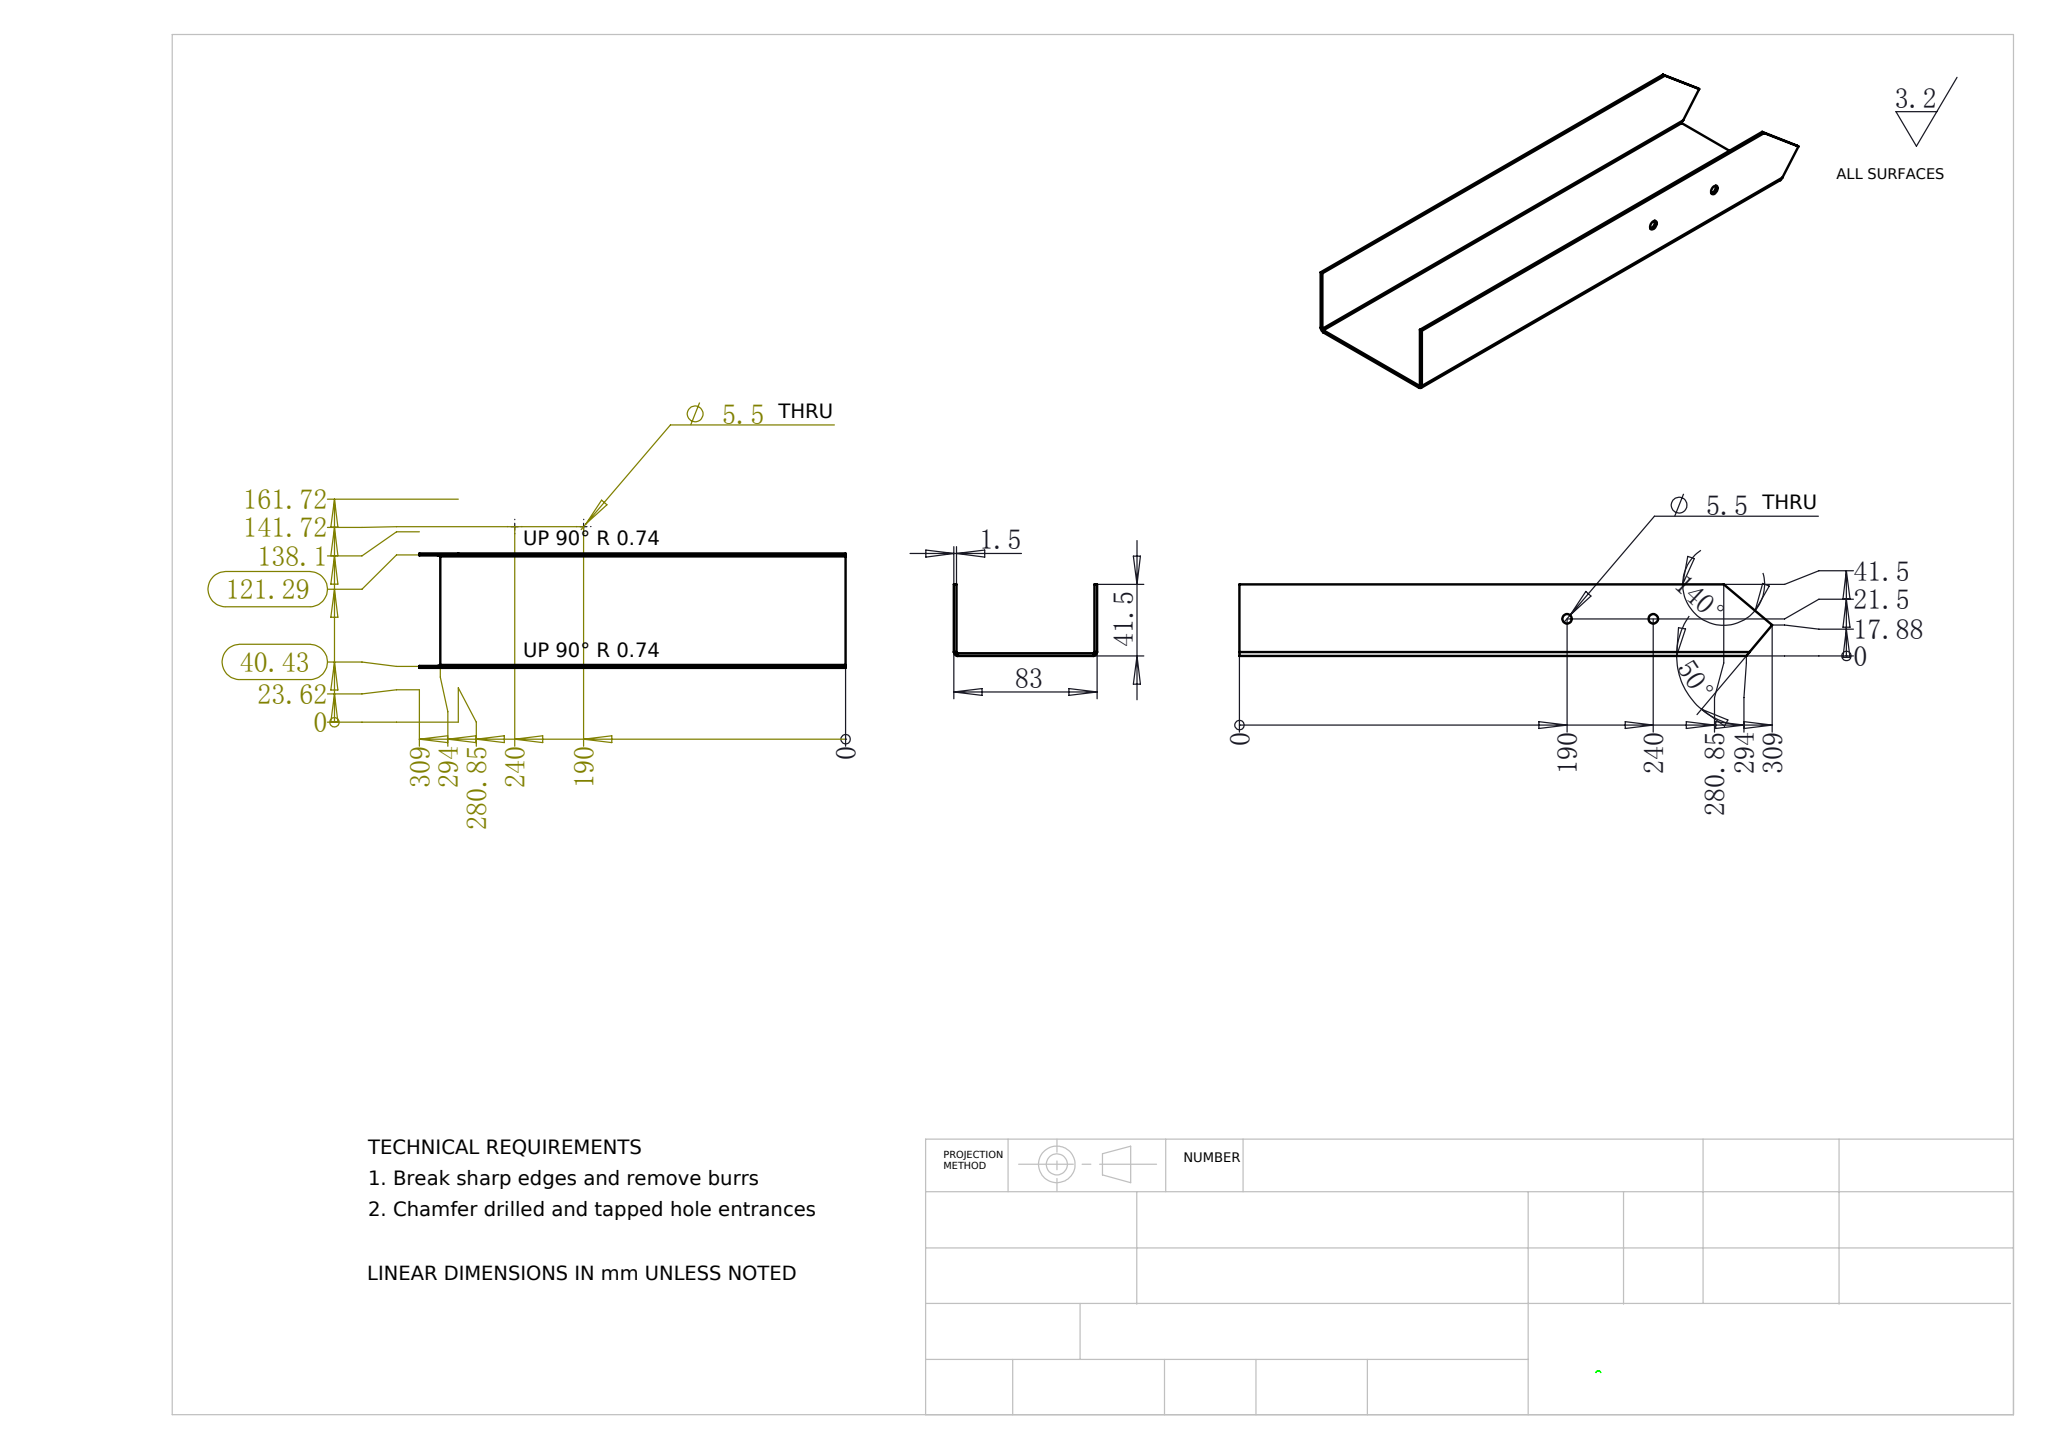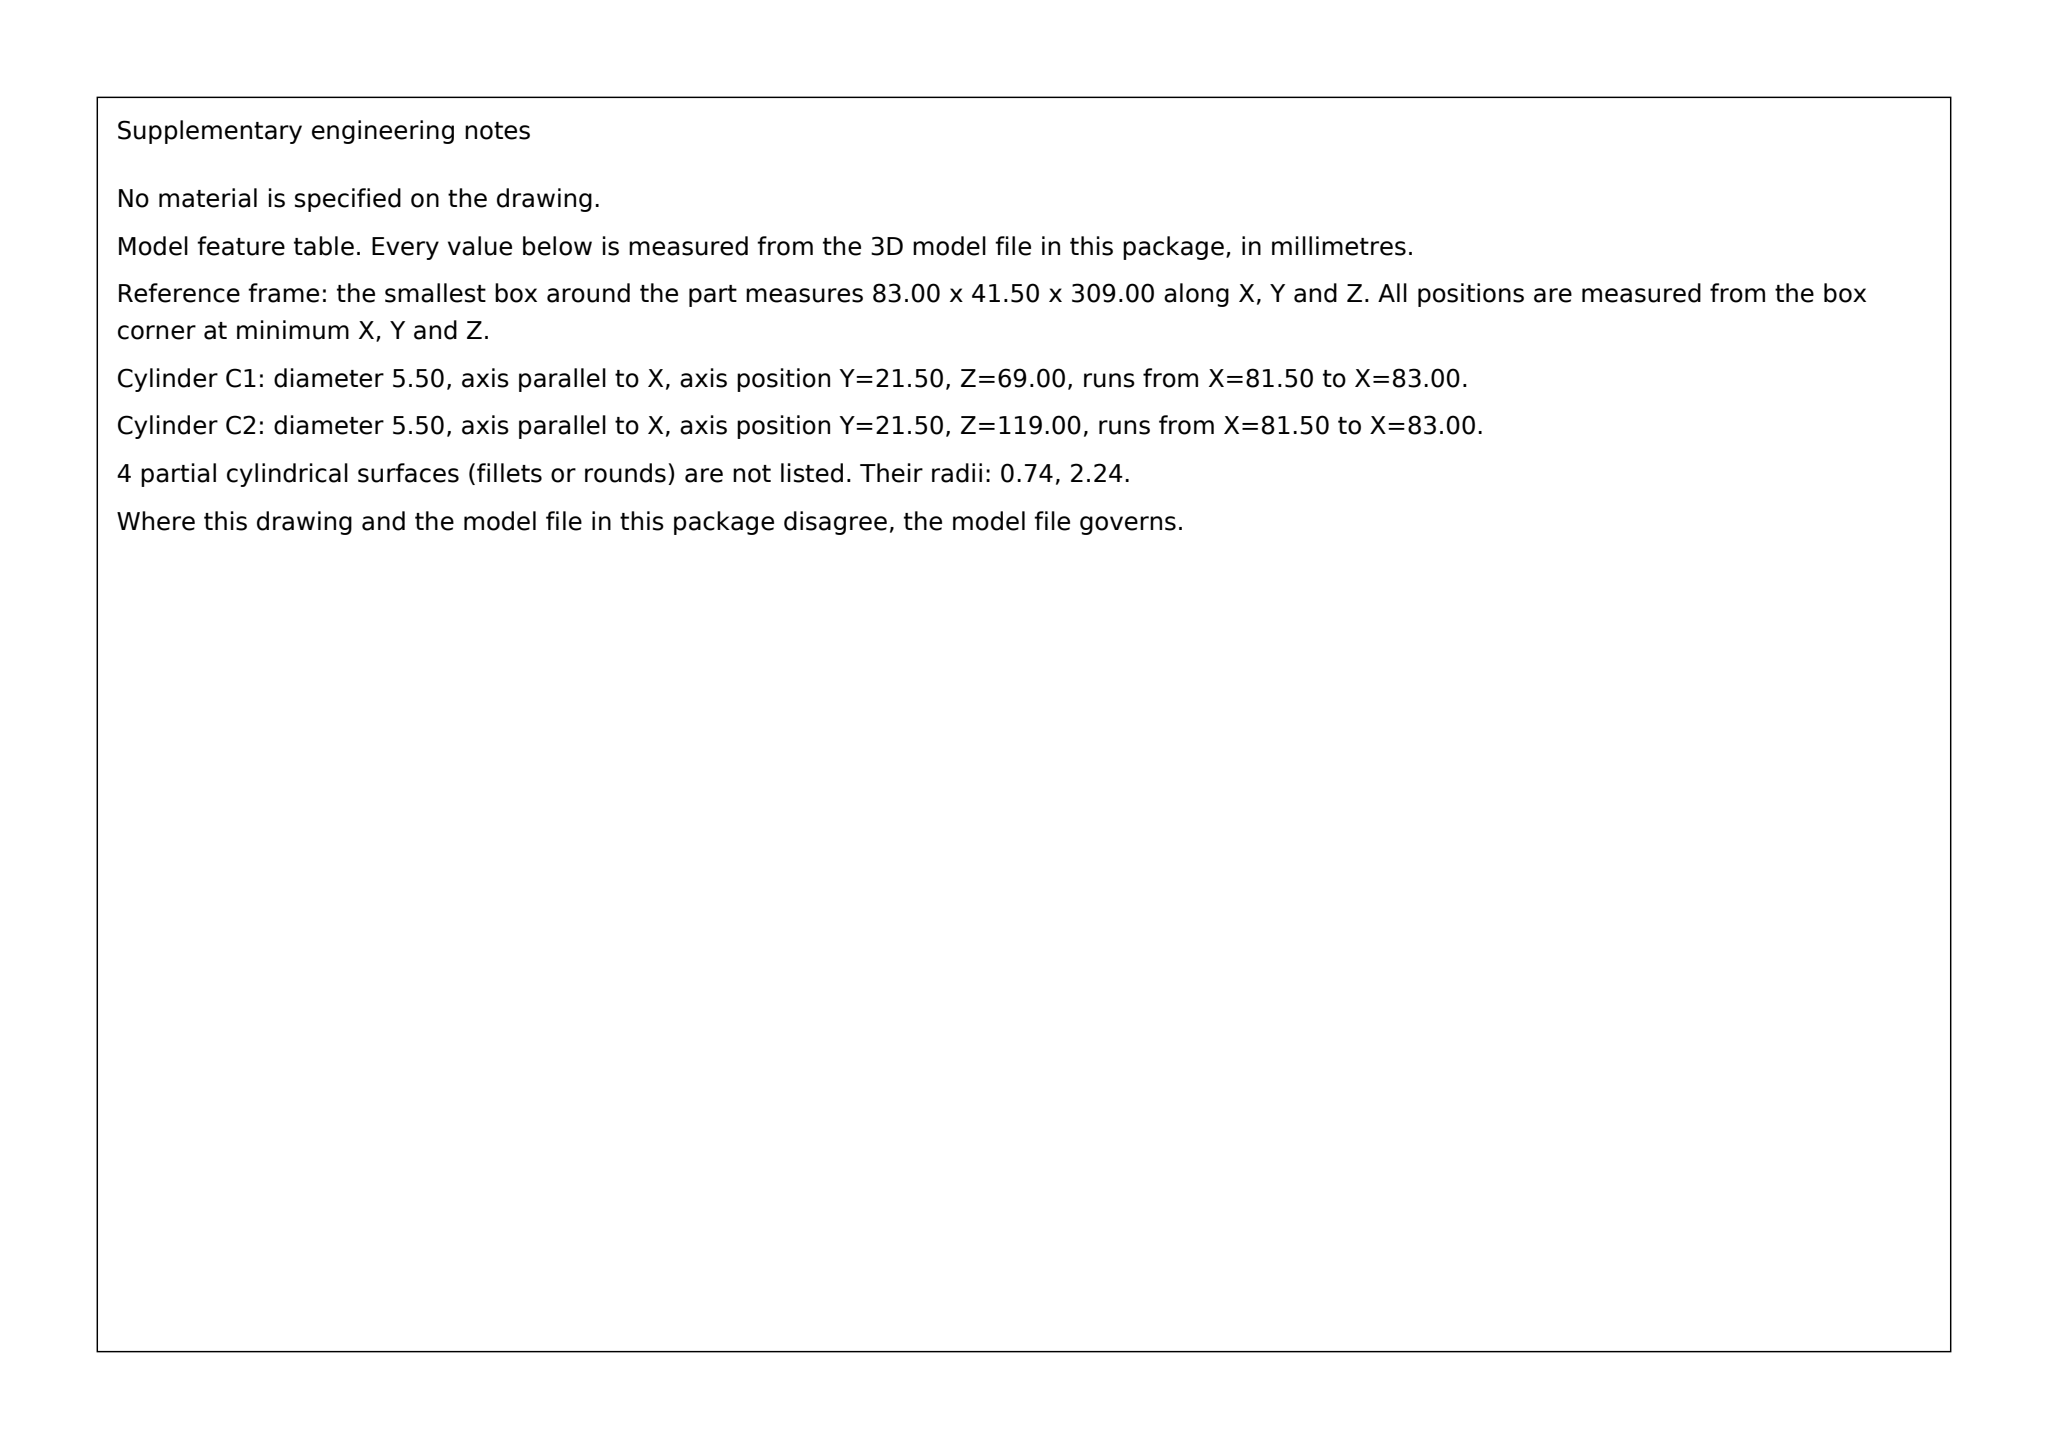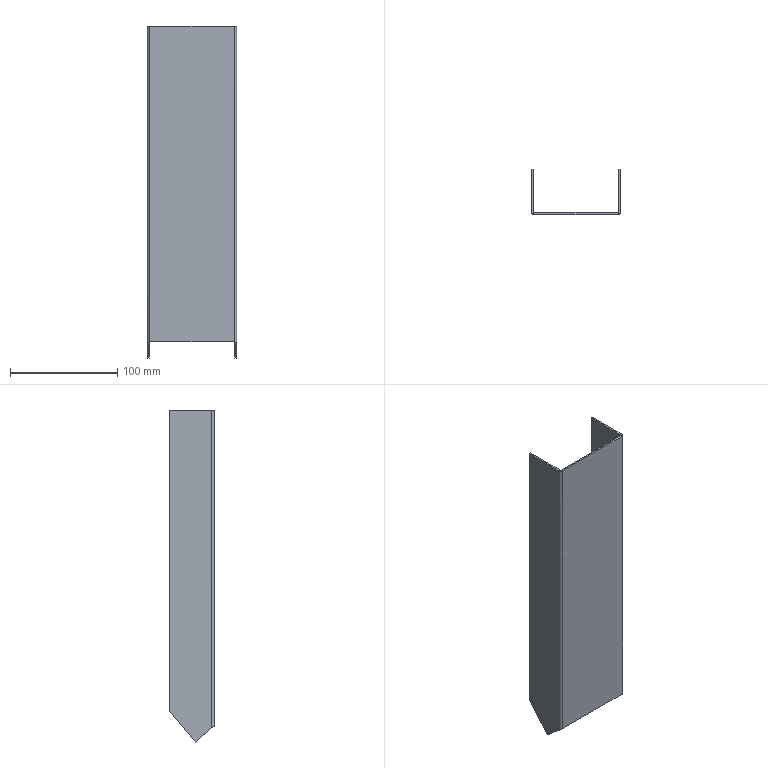Part | SolidWorks | mm | 1 solid | 28 faces | box 83 x 41.5 x 309 mm | volume 71715 mm3 | plane 18 | cylinder 8 | spline 2 | commonest cylinder face diameters 5.5 x4 1.473 x2 4.473 x2
STEP:
#1=CARTESIAN_POINT('',(80.,20.,-232.75));
#2=VERTEX_POINT('',#1);
#3=CARTESIAN_POINT('',(80.,20.,-227.25));
#4=VERTEX_POINT('',#3);
#5=CARTESIAN_POINT('',(80.,20.,-230.));
#6=DIRECTION('',(-1.,0.,0.));
#7=DIRECTION('',(0.,0.,1.));
#8=AXIS2_PLACEMENT_3D('',#5,#6,#7);
#9=CIRCLE('',#8,2.75);
#10=EDGE_CURVE('',#2,#4,#9,.T.);
#11=ORIENTED_EDGE('',*,*,#10,.T.);
#12=CARTESIAN_POINT('',(81.5,20.,-227.25));
#13=VERTEX_POINT('',#12);
#14=CARTESIAN_POINT('',(81.5,20.,-227.25));
#15=DIRECTION('',(1.,0.,0.));
#16=VECTOR('',#15,1000.);
#17=LINE('',#14,#16);
#18=EDGE_CURVE('',#4,#13,#17,.T.);
#19=ORIENTED_EDGE('',*,*,#18,.T.);
#20=CARTESIAN_POINT('',(81.5,20.,-232.75));
#21=VERTEX_POINT('',#20);
#22=CARTESIAN_POINT('',(81.5,20.,-230.));
#23=DIRECTION('',(1.,0.,0.));
#24=DIRECTION('',(0.,0.,-1.));
#25=AXIS2_PLACEMENT_3D('',#22,#23,#24);
#26=CIRCLE('',#25,2.75);
#27=EDGE_CURVE('',#13,#21,#26,.T.);
#28=ORIENTED_EDGE('',*,*,#27,.T.);
#29=CARTESIAN_POINT('',(81.5,20.,-232.75));
#30=DIRECTION('',(1.,0.,0.));
#31=VECTOR('',#30,1000.);
#32=LINE('',#29,#31);
#33=EDGE_CURVE('',#2,#21,#32,.T.);
#34=ORIENTED_EDGE('',*,*,#33,.F.);
#35=EDGE_LOOP('',(#11,#19,#28,#34));
#36=FACE_OUTER_BOUND('',#35,.T.);
#37=CARTESIAN_POINT('',(81.5,20.,-230.));
#38=DIRECTION('',(1.,0.,0.));
#39=DIRECTION('',(0.,0.,-1.));
#40=AXIS2_PLACEMENT_3D('',#37,#38,#39);
#41=CYLINDRICAL_SURFACE('',#40,2.75);
#42=ADVANCED_FACE('',(#36),#41,.F.);
#43=CARTESIAN_POINT('',(80.,20.,-182.75));
#44=VERTEX_POINT('',#43);
#45=CARTESIAN_POINT('',(80.,20.,-177.25));
#46=VERTEX_POINT('',#45);
#47=CARTESIAN_POINT('',(80.,20.,-180.));
#48=DIRECTION('',(-1.,0.,0.));
#49=DIRECTION('',(0.,0.,1.));
#50=AXIS2_PLACEMENT_3D('',#47,#48,#49);
#51=CIRCLE('',#50,2.75);
#52=EDGE_CURVE('',#44,#46,#51,.T.);
#53=ORIENTED_EDGE('',*,*,#52,.T.);
#54=CARTESIAN_POINT('',(81.5,20.,-177.25));
#55=VERTEX_POINT('',#54);
#56=CARTESIAN_POINT('',(81.5,20.,-177.25));
#57=DIRECTION('',(1.,0.,0.));
#58=VECTOR('',#57,1000.);
#59=LINE('',#56,#58);
#60=EDGE_CURVE('',#46,#55,#59,.T.);
#61=ORIENTED_EDGE('',*,*,#60,.T.);
#62=CARTESIAN_POINT('',(81.5,20.,-182.75));
#63=VERTEX_POINT('',#62);
#64=CARTESIAN_POINT('',(81.5,20.,-180.));
#65=DIRECTION('',(1.,0.,0.));
#66=DIRECTION('',(0.,0.,-1.));
#67=AXIS2_PLACEMENT_3D('',#64,#65,#66);
#68=CIRCLE('',#67,2.75);
#69=EDGE_CURVE('',#55,#63,#68,.T.);
#70=ORIENTED_EDGE('',*,*,#69,.T.);
#71=CARTESIAN_POINT('',(81.5,20.,-182.75));
#72=DIRECTION('',(1.,0.,0.));
#73=VECTOR('',#72,1000.);
#74=LINE('',#71,#73);
#75=EDGE_CURVE('',#44,#63,#74,.T.);
#76=ORIENTED_EDGE('',*,*,#75,.F.);
#77=EDGE_LOOP('',(#53,#61,#70,#76));
#78=FACE_OUTER_BOUND('',#77,.T.);
#79=CARTESIAN_POINT('',(81.5,20.,-180.));
#80=DIRECTION('',(1.,0.,0.));
#81=DIRECTION('',(0.,0.,-1.));
#82=AXIS2_PLACEMENT_3D('',#79,#80,#81);
#83=CYLINDRICAL_SURFACE('',#82,2.75);
#84=ADVANCED_FACE('',(#78),#83,.F.);
#85=CARTESIAN_POINT('',(81.5,20.,-230.));
#86=DIRECTION('',(1.,0.,0.));
#87=DIRECTION('',(0.,0.,-1.));
#88=AXIS2_PLACEMENT_3D('',#85,#86,#87);
#89=CIRCLE('',#88,2.75);
#90=EDGE_CURVE('',#21,#13,#89,.T.);
#91=ORIENTED_EDGE('',*,*,#90,.F.);
#92=ORIENTED_EDGE('',*,*,#27,.F.);
#93=EDGE_LOOP('',(#91,#92));
#94=FACE_BOUND('',#93,.T.);
#95=CARTESIAN_POINT('',(81.5,20.,-180.));
#96=DIRECTION('',(1.,0.,0.));
#97=DIRECTION('',(0.,0.,-1.));
#98=AXIS2_PLACEMENT_3D('',#95,#96,#97);
#99=CIRCLE('',#98,2.75);
#100=EDGE_CURVE('',#63,#55,#99,.T.);
#101=ORIENTED_EDGE('',*,*,#100,.F.);
#102=ORIENTED_EDGE('',*,*,#69,.F.);
#103=EDGE_LOOP('',(#101,#102));
#104=FACE_BOUND('',#103,.T.);
#105=CARTESIAN_POINT('',(81.5,0.7366,-285.877));
#106=VERTEX_POINT('',#105);
#107=CARTESIAN_POINT('',(81.5,16.376,-299.));
#108=VERTEX_POINT('',#107);
#109=CARTESIAN_POINT('',(81.5,-145.387,-163.265));
#110=DIRECTION('',(0.,0.766,-0.6428));
#111=VECTOR('',#110,1000.);
#112=LINE('',#109,#111);
#113=EDGE_CURVE('',#106,#108,#112,.T.);
#114=ORIENTED_EDGE('',*,*,#113,.T.);
#115=CARTESIAN_POINT('',(81.5,40.,-270.846));
#116=VERTEX_POINT('',#115);
#117=CARTESIAN_POINT('',(81.5,161.763,-125.735));
#118=DIRECTION('',(0.,0.6428,0.766));
#119=VECTOR('',#118,1000.);
#120=LINE('',#117,#119);
#121=EDGE_CURVE('',#108,#116,#120,.T.);
#122=ORIENTED_EDGE('',*,*,#121,.T.);
#123=CARTESIAN_POINT('',(81.5,40.,10.));
#124=VERTEX_POINT('',#123);
#125=CARTESIAN_POINT('',(81.5,40.,10.));
#126=DIRECTION('',(0.,0.,-1.));
#127=VECTOR('',#126,1000.);
#128=LINE('',#125,#127);
#129=EDGE_CURVE('',#124,#116,#128,.T.);
#130=ORIENTED_EDGE('',*,*,#129,.F.);
#131=CARTESIAN_POINT('',(81.5,0.7366,10.));
#132=VERTEX_POINT('',#131);
#133=CARTESIAN_POINT('',(81.5,0.,10.));
#134=DIRECTION('',(0.,1.,0.));
#135=VECTOR('',#134,1000.);
#136=LINE('',#133,#135);
#137=EDGE_CURVE('',#132,#124,#136,.T.);
#138=ORIENTED_EDGE('',*,*,#137,.F.);
#139=CARTESIAN_POINT('',(81.5,0.7366,10.));
#140=DIRECTION('',(0.,0.,-1.));
#141=VECTOR('',#140,1000.);
#142=LINE('',#139,#141);
#143=EDGE_CURVE('',#132,#106,#142,.T.);
#144=ORIENTED_EDGE('',*,*,#143,.T.);
#145=EDGE_LOOP('',(#114,#122,#130,#138,#144));
#146=FACE_OUTER_BOUND('',#145,.T.);
#147=CARTESIAN_POINT('',(81.5,0.,10.));
#148=DIRECTION('',(-1.,0.,0.));
#149=DIRECTION('',(0.,0.,1.));
#150=AXIS2_PLACEMENT_3D('',#147,#148,#149);
#151=PLANE('',#150);
#152=ADVANCED_FACE('',(#94,#104,#146),#151,.F.);
#153=ORIENTED_EDGE('',*,*,#129,.T.);
#154=CARTESIAN_POINT('',(80.,40.,-270.846));
#155=VERTEX_POINT('',#154);
#156=CARTESIAN_POINT('',(80.,40.,-270.846));
#157=DIRECTION('',(1.,0.,0.));
#158=VECTOR('',#157,1000.);
#159=LINE('',#156,#158);
#160=EDGE_CURVE('',#155,#116,#159,.T.);
#161=ORIENTED_EDGE('',*,*,#160,.F.);
#162=CARTESIAN_POINT('',(80.,40.,10.));
#163=VERTEX_POINT('',#162);
#164=CARTESIAN_POINT('',(80.,40.,10.));
#165=DIRECTION('',(0.,0.,-1.));
#166=VECTOR('',#165,1000.);
#167=LINE('',#164,#166);
#168=EDGE_CURVE('',#163,#155,#167,.T.);
#169=ORIENTED_EDGE('',*,*,#168,.F.);
#170=CARTESIAN_POINT('',(80.,40.,10.));
#171=DIRECTION('',(1.,0.,0.));
#172=VECTOR('',#171,1000.);
#173=LINE('',#170,#172);
#174=EDGE_CURVE('',#163,#124,#173,.T.);
#175=ORIENTED_EDGE('',*,*,#174,.T.);
#176=EDGE_LOOP('',(#153,#161,#169,#175));
#177=FACE_OUTER_BOUND('',#176,.T.);
#178=CARTESIAN_POINT('',(80.,40.,10.));
#179=DIRECTION('',(0.,1.,0.));
#180=DIRECTION('',(0.,0.,1.));
#181=AXIS2_PLACEMENT_3D('',#178,#179,#180);
#182=PLANE('',#181);
#183=ADVANCED_FACE('',(#177),#182,.T.);
#184=ORIENTED_EDGE('',*,*,#10,.F.);
#185=CARTESIAN_POINT('',(80.,20.,-230.));
#186=DIRECTION('',(-1.,0.,0.));
#187=DIRECTION('',(0.,0.,1.));
#188=AXIS2_PLACEMENT_3D('',#185,#186,#187);
#189=CIRCLE('',#188,2.75);
#190=EDGE_CURVE('',#4,#2,#189,.T.);
#191=ORIENTED_EDGE('',*,*,#190,.F.);
#192=EDGE_LOOP('',(#184,#191));
#193=FACE_BOUND('',#192,.T.);
#194=ORIENTED_EDGE('',*,*,#52,.F.);
#195=CARTESIAN_POINT('',(80.,20.,-180.));
#196=DIRECTION('',(-1.,0.,0.));
#197=DIRECTION('',(0.,0.,1.));
#198=AXIS2_PLACEMENT_3D('',#195,#196,#197);
#199=CIRCLE('',#198,2.75);
#200=EDGE_CURVE('',#46,#44,#199,.T.);
#201=ORIENTED_EDGE('',*,*,#200,.F.);
#202=EDGE_LOOP('',(#194,#201));
#203=FACE_BOUND('',#202,.T.);
#204=CARTESIAN_POINT('',(80.,16.376,-299.));
#205=VERTEX_POINT('',#204);
#206=CARTESIAN_POINT('',(80.,161.763,-125.735));
#207=DIRECTION('',(0.,0.6428,0.766));
#208=VECTOR('',#207,1000.);
#209=LINE('',#206,#208);
#210=EDGE_CURVE('',#205,#155,#209,.T.);
#211=ORIENTED_EDGE('',*,*,#210,.F.);
#212=CARTESIAN_POINT('',(80.,0.7366,-285.877));
#213=VERTEX_POINT('',#212);
#214=CARTESIAN_POINT('',(80.,-145.387,-163.265));
#215=DIRECTION('',(0.,0.766,-0.6428));
#216=VECTOR('',#215,1000.);
#217=LINE('',#214,#216);
#218=EDGE_CURVE('',#213,#205,#217,.T.);
#219=ORIENTED_EDGE('',*,*,#218,.F.);
#220=CARTESIAN_POINT('',(80.,0.7366,10.));
#221=VERTEX_POINT('',#220);
#222=CARTESIAN_POINT('',(80.,0.7366,10.));
#223=DIRECTION('',(0.,0.,-1.));
#224=VECTOR('',#223,1000.);
#225=LINE('',#222,#224);
#226=EDGE_CURVE('',#221,#213,#225,.T.);
#227=ORIENTED_EDGE('',*,*,#226,.F.);
#228=CARTESIAN_POINT('',(80.,0.,10.));
#229=DIRECTION('',(0.,1.,0.));
#230=VECTOR('',#229,1000.);
#231=LINE('',#228,#230);
#232=EDGE_CURVE('',#221,#163,#231,.T.);
#233=ORIENTED_EDGE('',*,*,#232,.T.);
#234=ORIENTED_EDGE('',*,*,#168,.T.);
#235=EDGE_LOOP('',(#211,#219,#227,#233,#234));
#236=FACE_OUTER_BOUND('',#235,.T.);
#237=CARTESIAN_POINT('',(80.,0.,10.));
#238=DIRECTION('',(-1.,0.,0.));
#239=DIRECTION('',(0.,0.,1.));
#240=AXIS2_PLACEMENT_3D('',#237,#238,#239);
#241=PLANE('',#240);
#242=ADVANCED_FACE('',(#193,#203,#236),#241,.T.);
#243=ORIENTED_EDGE('',*,*,#226,.T.);
#244=CARTESIAN_POINT('',(79.263,0.,-284.));
#245=VERTEX_POINT('',#244);
#246=CARTESIAN_POINT('',(79.263,0.,-284.));
#247=CARTESIAN_POINT('',(79.695,-0.,-284.));
#248=CARTESIAN_POINT('',(80.,0.3051,-284.777));
#249=CARTESIAN_POINT('',(80.,0.7366,-285.877));
#250=(BOUNDED_CURVE()B_SPLINE_CURVE(3,(#246,#247,#248,#249),.UNSPECIFIED.,.F.,.F.)B_SPLINE_CURVE_WITH_KNOTS((4,4),(3.142,4.712),.UNSPECIFIED.)CURVE()GEOMETRIC_REPRESENTATION_ITEM()RATIONAL_B_SPLINE_CURVE((1.,0.8047,0.8047,1.))REPRESENTATION_ITEM(''));
#251=EDGE_CURVE('',#245,#213,#250,.T.);
#252=ORIENTED_EDGE('',*,*,#251,.F.);
#253=CARTESIAN_POINT('',(79.263,0.,10.));
#254=VERTEX_POINT('',#253);
#255=CARTESIAN_POINT('',(79.263,0.,10.));
#256=DIRECTION('',(0.,0.,-1.));
#257=VECTOR('',#256,1000.);
#258=LINE('',#255,#257);
#259=EDGE_CURVE('',#254,#245,#258,.T.);
#260=ORIENTED_EDGE('',*,*,#259,.F.);
#261=CARTESIAN_POINT('',(79.263,0.7366,10.));
#262=DIRECTION('',(0.,0.,1.));
#263=DIRECTION('',(-1.,0.,0.));
#264=AXIS2_PLACEMENT_3D('',#261,#262,#263);
#265=CIRCLE('',#264,0.7366);
#266=EDGE_CURVE('',#254,#221,#265,.T.);
#267=ORIENTED_EDGE('',*,*,#266,.T.);
#268=EDGE_LOOP('',(#243,#252,#260,#267));
#269=FACE_OUTER_BOUND('',#268,.T.);
#270=CARTESIAN_POINT('',(79.263,0.7366,10.));
#271=DIRECTION('',(0.,0.,-1.));
#272=DIRECTION('',(-1.,0.,0.));
#273=AXIS2_PLACEMENT_3D('',#270,#271,#272);
#274=CYLINDRICAL_SURFACE('',#273,0.7366);
#275=ADVANCED_FACE('',(#269),#274,.F.);
#276=ORIENTED_EDGE('',*,*,#259,.T.);
#277=CARTESIAN_POINT('',(0.7366,0.,-284.));
#278=VERTEX_POINT('',#277);
#279=CARTESIAN_POINT('',(0.,0.,-284.));
#280=DIRECTION('',(-1.,0.,0.));
#281=VECTOR('',#280,1000.);
#282=LINE('',#279,#281);
#283=EDGE_CURVE('',#245,#278,#282,.T.);
#284=ORIENTED_EDGE('',*,*,#283,.T.);
#285=CARTESIAN_POINT('',(0.7366,0.,10.));
#286=VERTEX_POINT('',#285);
#287=CARTESIAN_POINT('',(0.7366,0.,10.));
#288=DIRECTION('',(0.,0.,-1.));
#289=VECTOR('',#288,1000.);
#290=LINE('',#287,#289);
#291=EDGE_CURVE('',#286,#278,#290,.T.);
#292=ORIENTED_EDGE('',*,*,#291,.F.);
#293=CARTESIAN_POINT('',(0.,0.,10.));
#294=DIRECTION('',(1.,0.,0.));
#295=VECTOR('',#294,1000.);
#296=LINE('',#293,#295);
#297=EDGE_CURVE('',#286,#254,#296,.T.);
#298=ORIENTED_EDGE('',*,*,#297,.T.);
#299=EDGE_LOOP('',(#276,#284,#292,#298));
#300=FACE_OUTER_BOUND('',#299,.T.);
#301=CARTESIAN_POINT('',(0.,0.,10.));
#302=DIRECTION('',(0.,1.,0.));
#303=DIRECTION('',(0.,0.,1.));
#304=AXIS2_PLACEMENT_3D('',#301,#302,#303);
#305=PLANE('',#304);
#306=ADVANCED_FACE('',(#300),#305,.T.);
#307=ORIENTED_EDGE('',*,*,#291,.T.);
#308=CARTESIAN_POINT('',(0.,0.7366,-285.877));
#309=VERTEX_POINT('',#308);
#310=CARTESIAN_POINT('',(0.,0.7366,-285.877));
#311=CARTESIAN_POINT('',(-0.,0.3051,-284.777));
#312=CARTESIAN_POINT('',(0.3051,-0.,-284.));
#313=CARTESIAN_POINT('',(0.7366,0.,-284.));
#314=(BOUNDED_CURVE()B_SPLINE_CURVE(3,(#310,#311,#312,#313),.UNSPECIFIED.,.F.,.F.)B_SPLINE_CURVE_WITH_KNOTS((4,4),(1.571,3.142),.UNSPECIFIED.)CURVE()GEOMETRIC_REPRESENTATION_ITEM()RATIONAL_B_SPLINE_CURVE((1.,0.8047,0.8047,1.))REPRESENTATION_ITEM(''));
#315=EDGE_CURVE('',#309,#278,#314,.T.);
#316=ORIENTED_EDGE('',*,*,#315,.F.);
#317=CARTESIAN_POINT('',(0.,0.7366,10.));
#318=VERTEX_POINT('',#317);
#319=CARTESIAN_POINT('',(0.,0.7366,10.));
#320=DIRECTION('',(0.,0.,-1.));
#321=VECTOR('',#320,1000.);
#322=LINE('',#319,#321);
#323=EDGE_CURVE('',#318,#309,#322,.T.);
#324=ORIENTED_EDGE('',*,*,#323,.F.);
#325=CARTESIAN_POINT('',(0.7366,0.7366,10.));
#326=DIRECTION('',(0.,0.,1.));
#327=DIRECTION('',(-1.,0.,0.));
#328=AXIS2_PLACEMENT_3D('',#325,#326,#327);
#329=CIRCLE('',#328,0.7366);
#330=EDGE_CURVE('',#318,#286,#329,.T.);
#331=ORIENTED_EDGE('',*,*,#330,.T.);
#332=EDGE_LOOP('',(#307,#316,#324,#331));
#333=FACE_OUTER_BOUND('',#332,.T.);
#334=CARTESIAN_POINT('',(0.7366,0.7366,10.));
#335=DIRECTION('',(0.,0.,-1.));
#336=DIRECTION('',(-1.,0.,0.));
#337=AXIS2_PLACEMENT_3D('',#334,#335,#336);
#338=CYLINDRICAL_SURFACE('',#337,0.7366);
#339=ADVANCED_FACE('',(#333),#338,.F.);
#340=CARTESIAN_POINT('',(0.,16.376,-299.));
#341=VERTEX_POINT('',#340);
#342=CARTESIAN_POINT('',(0.,-145.387,-163.265));
#343=DIRECTION('',(0.,-0.766,0.6428));
#344=VECTOR('',#343,1000.);
#345=LINE('',#342,#344);
#346=EDGE_CURVE('',#341,#309,#345,.T.);
#347=ORIENTED_EDGE('',*,*,#346,.F.);
#348=CARTESIAN_POINT('',(0.,40.,-270.846));
#349=VERTEX_POINT('',#348);
#350=CARTESIAN_POINT('',(0.,161.763,-125.735));
#351=DIRECTION('',(0.,-0.6428,-0.766));
#352=VECTOR('',#351,1000.);
#353=LINE('',#350,#352);
#354=EDGE_CURVE('',#349,#341,#353,.T.);
#355=ORIENTED_EDGE('',*,*,#354,.F.);
#356=CARTESIAN_POINT('',(0.,40.,10.));
#357=VERTEX_POINT('',#356);
#358=CARTESIAN_POINT('',(0.,40.,10.));
#359=DIRECTION('',(0.,0.,-1.));
#360=VECTOR('',#359,1000.);
#361=LINE('',#358,#360);
#362=EDGE_CURVE('',#357,#349,#361,.T.);
#363=ORIENTED_EDGE('',*,*,#362,.F.);
#364=CARTESIAN_POINT('',(0.,0.,10.));
#365=DIRECTION('',(0.,-1.,0.));
#366=VECTOR('',#365,1000.);
#367=LINE('',#364,#366);
#368=EDGE_CURVE('',#357,#318,#367,.T.);
#369=ORIENTED_EDGE('',*,*,#368,.T.);
#370=ORIENTED_EDGE('',*,*,#323,.T.);
#371=EDGE_LOOP('',(#347,#355,#363,#369,#370));
#372=FACE_OUTER_BOUND('',#371,.T.);
#373=CARTESIAN_POINT('',(0.,0.,10.));
#374=DIRECTION('',(1.,0.,0.));
#375=DIRECTION('',(0.,0.,-1.));
#376=AXIS2_PLACEMENT_3D('',#373,#374,#375);
#377=PLANE('',#376);
#378=ADVANCED_FACE('',(#372),#377,.T.);
#379=ORIENTED_EDGE('',*,*,#362,.T.);
#380=CARTESIAN_POINT('',(-1.5,40.,-270.846));
#381=VERTEX_POINT('',#380);
#382=CARTESIAN_POINT('',(0.,40.,-270.846));
#383=DIRECTION('',(-1.,0.,0.));
#384=VECTOR('',#383,1000.);
#385=LINE('',#382,#384);
#386=EDGE_CURVE('',#349,#381,#385,.T.);
#387=ORIENTED_EDGE('',*,*,#386,.T.);
#388=CARTESIAN_POINT('',(-1.5,40.,10.));
#389=VERTEX_POINT('',#388);
#390=CARTESIAN_POINT('',(-1.5,40.,10.));
#391=DIRECTION('',(0.,0.,-1.));
#392=VECTOR('',#391,1000.);
#393=LINE('',#390,#392);
#394=EDGE_CURVE('',#389,#381,#393,.T.);
#395=ORIENTED_EDGE('',*,*,#394,.F.);
#396=CARTESIAN_POINT('',(-1.5,40.,10.));
#397=DIRECTION('',(1.,0.,0.));
#398=VECTOR('',#397,1000.);
#399=LINE('',#396,#398);
#400=EDGE_CURVE('',#389,#357,#399,.T.);
#401=ORIENTED_EDGE('',*,*,#400,.T.);
#402=EDGE_LOOP('',(#379,#387,#395,#401));
#403=FACE_OUTER_BOUND('',#402,.T.);
#404=CARTESIAN_POINT('',(-1.5,40.,10.));
#405=DIRECTION('',(0.,1.,0.));
#406=DIRECTION('',(0.,0.,1.));
#407=AXIS2_PLACEMENT_3D('',#404,#405,#406);
#408=PLANE('',#407);
#409=ADVANCED_FACE('',(#403),#408,.T.);
#410=CARTESIAN_POINT('',(-1.5,16.376,-299.));
#411=VERTEX_POINT('',#410);
#412=CARTESIAN_POINT('',(-1.5,161.763,-125.735));
#413=DIRECTION('',(0.,-0.6428,-0.766));
#414=VECTOR('',#413,1000.);
#415=LINE('',#412,#414);
#416=EDGE_CURVE('',#381,#411,#415,.T.);
#417=ORIENTED_EDGE('',*,*,#416,.T.);
#418=CARTESIAN_POINT('',(-1.5,0.7366,-285.877));
#419=VERTEX_POINT('',#418);
#420=CARTESIAN_POINT('',(-1.5,-145.387,-163.265));
#421=DIRECTION('',(0.,-0.766,0.6428));
#422=VECTOR('',#421,1000.);
#423=LINE('',#420,#422);
#424=EDGE_CURVE('',#411,#419,#423,.T.);
#425=ORIENTED_EDGE('',*,*,#424,.T.);
#426=CARTESIAN_POINT('',(-1.5,0.7366,10.));
#427=VERTEX_POINT('',#426);
#428=CARTESIAN_POINT('',(-1.5,0.7366,10.));
#429=DIRECTION('',(0.,0.,-1.));
#430=VECTOR('',#429,1000.);
#431=LINE('',#428,#430);
#432=EDGE_CURVE('',#427,#419,#431,.T.);
#433=ORIENTED_EDGE('',*,*,#432,.F.);
#434=CARTESIAN_POINT('',(-1.5,0.,10.));
#435=DIRECTION('',(0.,-1.,0.));
#436=VECTOR('',#435,1000.);
#437=LINE('',#434,#436);
#438=EDGE_CURVE('',#389,#427,#437,.T.);
#439=ORIENTED_EDGE('',*,*,#438,.F.);
#440=ORIENTED_EDGE('',*,*,#394,.T.);
#441=EDGE_LOOP('',(#417,#425,#433,#439,#440));
#442=FACE_OUTER_BOUND('',#441,.T.);
#443=CARTESIAN_POINT('',(-1.5,0.,10.));
#444=DIRECTION('',(1.,0.,0.));
#445=DIRECTION('',(0.,0.,-1.));
#446=AXIS2_PLACEMENT_3D('',#443,#444,#445);
#447=PLANE('',#446);
#448=ADVANCED_FACE('',(#442),#447,.F.);
#449=CARTESIAN_POINT('',(0.7366,-1.5,-284.));
#450=VERTEX_POINT('',#449);
#451=CARTESIAN_POINT('',(-1.5,0.7366,-285.877));
#452=CARTESIAN_POINT('',(-1.5,-0.5736,-284.777));
#453=CARTESIAN_POINT('',(-0.5736,-1.5,-284.));
#454=CARTESIAN_POINT('',(0.7366,-1.5,-284.));
#455=(BOUNDED_CURVE()B_SPLINE_CURVE(3,(#451,#452,#453,#454),.UNSPECIFIED.,.F.,.F.)B_SPLINE_CURVE_WITH_KNOTS((4,4),(1.571,3.142),.UNSPECIFIED.)CURVE()GEOMETRIC_REPRESENTATION_ITEM()RATIONAL_B_SPLINE_CURVE((1.,0.8047,0.8047,1.))REPRESENTATION_ITEM(''));
#456=EDGE_CURVE('',#419,#450,#455,.T.);
#457=ORIENTED_EDGE('',*,*,#456,.T.);
#458=CARTESIAN_POINT('',(0.7366,-1.5,10.));
#459=VERTEX_POINT('',#458);
#460=CARTESIAN_POINT('',(0.7366,-1.5,10.));
#461=DIRECTION('',(0.,0.,-1.));
#462=VECTOR('',#461,1000.);
#463=LINE('',#460,#462);
#464=EDGE_CURVE('',#459,#450,#463,.T.);
#465=ORIENTED_EDGE('',*,*,#464,.F.);
#466=CARTESIAN_POINT('',(0.7366,0.7366,10.));
#467=DIRECTION('',(0.,0.,1.));
#468=DIRECTION('',(1.,0.,0.));
#469=AXIS2_PLACEMENT_3D('',#466,#467,#468);
#470=CIRCLE('',#469,2.237);
#471=EDGE_CURVE('',#427,#459,#470,.T.);
#472=ORIENTED_EDGE('',*,*,#471,.F.);
#473=ORIENTED_EDGE('',*,*,#432,.T.);
#474=EDGE_LOOP('',(#457,#465,#472,#473));
#475=FACE_OUTER_BOUND('',#474,.T.);
#476=CARTESIAN_POINT('',(0.7366,0.7366,10.));
#477=DIRECTION('',(0.,0.,-1.));
#478=DIRECTION('',(-1.,0.,0.));
#479=AXIS2_PLACEMENT_3D('',#476,#477,#478);
#480=CYLINDRICAL_SURFACE('',#479,2.237);
#481=ADVANCED_FACE('',(#475),#480,.T.);
#482=CARTESIAN_POINT('',(79.263,-1.5,-284.));
#483=VERTEX_POINT('',#482);
#484=CARTESIAN_POINT('',(81.5,-1.5,-284.));
#485=DIRECTION('',(-1.,0.,0.));
#486=VECTOR('',#485,1000.);
#487=LINE('',#484,#486);
#488=EDGE_CURVE('',#483,#450,#487,.T.);
#489=ORIENTED_EDGE('',*,*,#488,.F.);
#490=CARTESIAN_POINT('',(79.263,-1.5,10.));
#491=VERTEX_POINT('',#490);
#492=CARTESIAN_POINT('',(79.263,-1.5,10.));
#493=DIRECTION('',(0.,0.,-1.));
#494=VECTOR('',#493,1000.);
#495=LINE('',#492,#494);
#496=EDGE_CURVE('',#491,#483,#495,.T.);
#497=ORIENTED_EDGE('',*,*,#496,.F.);
#498=CARTESIAN_POINT('',(0.,-1.5,10.));
#499=DIRECTION('',(1.,0.,0.));
#500=VECTOR('',#499,1000.);
#501=LINE('',#498,#500);
#502=EDGE_CURVE('',#459,#491,#501,.T.);
#503=ORIENTED_EDGE('',*,*,#502,.F.);
#504=ORIENTED_EDGE('',*,*,#464,.T.);
#505=EDGE_LOOP('',(#489,#497,#503,#504));
#506=FACE_OUTER_BOUND('',#505,.T.);
#507=CARTESIAN_POINT('',(0.,-1.5,10.));
#508=DIRECTION('',(0.,1.,0.));
#509=DIRECTION('',(0.,0.,1.));
#510=AXIS2_PLACEMENT_3D('',#507,#508,#509);
#511=PLANE('',#510);
#512=ADVANCED_FACE('',(#506),#511,.F.);
#513=CARTESIAN_POINT('',(79.263,-1.5,-284.));
#514=CARTESIAN_POINT('',(80.574,-1.5,-284.));
#515=CARTESIAN_POINT('',(81.5,-0.5736,-284.777));
#516=CARTESIAN_POINT('',(81.5,0.7366,-285.877));
#517=(BOUNDED_CURVE()B_SPLINE_CURVE(3,(#513,#514,#515,#516),.UNSPECIFIED.,.F.,.F.)B_SPLINE_CURVE_WITH_KNOTS((4,4),(3.142,4.712),.UNSPECIFIED.)CURVE()GEOMETRIC_REPRESENTATION_ITEM()RATIONAL_B_SPLINE_CURVE((1.,0.8047,0.8047,1.))REPRESENTATION_ITEM(''));
#518=EDGE_CURVE('',#483,#106,#517,.T.);
#519=ORIENTED_EDGE('',*,*,#518,.T.);
#520=ORIENTED_EDGE('',*,*,#143,.F.);
#521=CARTESIAN_POINT('',(79.263,0.7366,10.));
#522=DIRECTION('',(0.,0.,1.));
#523=DIRECTION('',(1.,0.,0.));
#524=AXIS2_PLACEMENT_3D('',#521,#522,#523);
#525=CIRCLE('',#524,2.237);
#526=EDGE_CURVE('',#491,#132,#525,.T.);
#527=ORIENTED_EDGE('',*,*,#526,.F.);
#528=ORIENTED_EDGE('',*,*,#496,.T.);
#529=EDGE_LOOP('',(#519,#520,#527,#528));
#530=FACE_OUTER_BOUND('',#529,.T.);
#531=CARTESIAN_POINT('',(79.263,0.7366,10.));
#532=DIRECTION('',(0.,0.,-1.));
#533=DIRECTION('',(-1.,0.,0.));
#534=AXIS2_PLACEMENT_3D('',#531,#532,#533);
#535=CYLINDRICAL_SURFACE('',#534,2.237);
#536=ADVANCED_FACE('',(#530),#535,.T.);
#537=CARTESIAN_POINT('',(0.7366,0.,10.));
#538=DIRECTION('',(0.,-1.,0.));
#539=VECTOR('',#538,1000.);
#540=LINE('',#537,#539);
#541=EDGE_CURVE('',#286,#459,#540,.T.);
#542=ORIENTED_EDGE('',*,*,#541,.F.);
#543=ORIENTED_EDGE('',*,*,#330,.F.);
#544=CARTESIAN_POINT('',(-1.5,0.7366,10.));
#545=DIRECTION('',(1.,-0.,0.));
#546=VECTOR('',#545,1000.);
#547=LINE('',#544,#546);
#548=EDGE_CURVE('',#427,#318,#547,.T.);
#549=ORIENTED_EDGE('',*,*,#548,.F.);
#550=ORIENTED_EDGE('',*,*,#471,.T.);
#551=EDGE_LOOP('',(#542,#543,#549,#550));
#552=FACE_OUTER_BOUND('',#551,.T.);
#553=CARTESIAN_POINT('',(0.7366,0.,10.));
#554=DIRECTION('',(0.,0.,1.));
#555=DIRECTION('',(1.,0.,0.));
#556=AXIS2_PLACEMENT_3D('',#553,#554,#555);
#557=PLANE('',#556);
#558=ADVANCED_FACE('',(#552),#557,.T.);
#559=ORIENTED_EDGE('',*,*,#297,.F.);
#560=ORIENTED_EDGE('',*,*,#541,.T.);
#561=ORIENTED_EDGE('',*,*,#502,.T.);
#562=CARTESIAN_POINT('',(79.263,-1.5,10.));
#563=DIRECTION('',(0.,1.,0.));
#564=VECTOR('',#563,1000.);
#565=LINE('',#562,#564);
#566=EDGE_CURVE('',#491,#254,#565,.T.);
#567=ORIENTED_EDGE('',*,*,#566,.T.);
#568=EDGE_LOOP('',(#559,#560,#561,#567));
#569=FACE_OUTER_BOUND('',#568,.T.);
#570=CARTESIAN_POINT('',(-1.5,0.7366,10.));
#571=DIRECTION('',(0.,0.,1.));
#572=DIRECTION('',(1.,0.,0.));
#573=AXIS2_PLACEMENT_3D('',#570,#571,#572);
#574=PLANE('',#573);
#575=ADVANCED_FACE('',(#569),#574,.T.);
#576=CARTESIAN_POINT('',(80.,0.7366,10.));
#577=DIRECTION('',(1.,0.,0.));
#578=VECTOR('',#577,1000.);
#579=LINE('',#576,#578);
#580=EDGE_CURVE('',#221,#132,#579,.T.);
#581=ORIENTED_EDGE('',*,*,#580,.F.);
#582=ORIENTED_EDGE('',*,*,#266,.F.);
#583=ORIENTED_EDGE('',*,*,#566,.F.);
#584=ORIENTED_EDGE('',*,*,#526,.T.);
#585=EDGE_LOOP('',(#581,#582,#583,#584));
#586=FACE_OUTER_BOUND('',#585,.T.);
#587=CARTESIAN_POINT('',(80.,0.7366,10.));
#588=DIRECTION('',(0.,0.,1.));
#589=DIRECTION('',(1.,0.,0.));
#590=AXIS2_PLACEMENT_3D('',#587,#588,#589);
#591=PLANE('',#590);
#592=ADVANCED_FACE('',(#586),#591,.T.);
#593=ORIENTED_EDGE('',*,*,#232,.F.);
#594=ORIENTED_EDGE('',*,*,#580,.T.);
#595=ORIENTED_EDGE('',*,*,#137,.T.);
#596=ORIENTED_EDGE('',*,*,#174,.F.);
#597=EDGE_LOOP('',(#593,#594,#595,#596));
#598=FACE_OUTER_BOUND('',#597,.T.);
#599=CARTESIAN_POINT('',(79.263,-1.5,10.));
#600=DIRECTION('',(0.,0.,1.));
#601=DIRECTION('',(1.,0.,0.));
#602=AXIS2_PLACEMENT_3D('',#599,#600,#601);
#603=PLANE('',#602);
#604=ADVANCED_FACE('',(#598),#603,.T.);
#605=ORIENTED_EDGE('',*,*,#438,.T.);
#606=ORIENTED_EDGE('',*,*,#548,.T.);
#607=ORIENTED_EDGE('',*,*,#368,.F.);
#608=ORIENTED_EDGE('',*,*,#400,.F.);
#609=EDGE_LOOP('',(#605,#606,#607,#608));
#610=FACE_OUTER_BOUND('',#609,.T.);
#611=CARTESIAN_POINT('',(79.263,0.7366,10.));
#612=DIRECTION('',(0.,0.,-1.));
#613=DIRECTION('',(-1.,0.,0.));
#614=AXIS2_PLACEMENT_3D('',#611,#612,#613);
#615=PLANE('',#614);
#616=ADVANCED_FACE('',(#610),#615,.F.);
#617=CARTESIAN_POINT('',(80.,0.7366,-285.877));
#618=DIRECTION('',(1.,0.,0.));
#619=VECTOR('',#618,1000.);
#620=LINE('',#617,#619);
#621=EDGE_CURVE('',#213,#106,#620,.T.);
#622=ORIENTED_EDGE('',*,*,#621,.F.);
#623=ORIENTED_EDGE('',*,*,#218,.T.);
#624=CARTESIAN_POINT('',(80.,16.376,-299.));
#625=DIRECTION('',(1.,0.,0.));
#626=VECTOR('',#625,1000.);
#627=LINE('',#624,#626);
#628=EDGE_CURVE('',#205,#108,#627,.T.);
#629=ORIENTED_EDGE('',*,*,#628,.T.);
#630=ORIENTED_EDGE('',*,*,#113,.F.);
#631=EDGE_LOOP('',(#622,#623,#629,#630));
#632=FACE_OUTER_BOUND('',#631,.T.);
#633=CARTESIAN_POINT('',(80.,-145.387,-163.265));
#634=DIRECTION('',(0.,0.6428,0.766));
#635=DIRECTION('',(0.,0.766,-0.6428));
#636=AXIS2_PLACEMENT_3D('',#633,#634,#635);
#637=PLANE('',#636);
#638=ADVANCED_FACE('',(#632),#637,.F.);
#639=ORIENTED_EDGE('',*,*,#210,.T.);
#640=ORIENTED_EDGE('',*,*,#160,.T.);
#641=ORIENTED_EDGE('',*,*,#121,.F.);
#642=ORIENTED_EDGE('',*,*,#628,.F.);
#643=EDGE_LOOP('',(#639,#640,#641,#642));
#644=FACE_OUTER_BOUND('',#643,.T.);
#645=CARTESIAN_POINT('',(80.,161.763,-125.735));
#646=DIRECTION('',(0.,-0.766,0.6428));
#647=DIRECTION('',(0.,0.6428,0.766));
#648=AXIS2_PLACEMENT_3D('',#645,#646,#647);
#649=PLANE('',#648);
#650=ADVANCED_FACE('',(#644),#649,.F.);
#651=CARTESIAN_POINT('',(79.263,-1.5,-284.));
#652=DIRECTION('',(0.,1.,0.));
#653=VECTOR('',#652,1000.);
#654=LINE('',#651,#653);
#655=EDGE_CURVE('',#483,#245,#654,.T.);
#656=ORIENTED_EDGE('',*,*,#655,.F.);
#657=ORIENTED_EDGE('',*,*,#488,.T.);
#658=CARTESIAN_POINT('',(0.7366,-1.5,-284.));
#659=DIRECTION('',(0.,1.,0.));
#660=VECTOR('',#659,1000.);
#661=LINE('',#658,#660);
#662=EDGE_CURVE('',#450,#278,#661,.T.);
#663=ORIENTED_EDGE('',*,*,#662,.T.);
#664=ORIENTED_EDGE('',*,*,#283,.F.);
#665=EDGE_LOOP('',(#656,#657,#663,#664));
#666=FACE_OUTER_BOUND('',#665,.T.);
#667=CARTESIAN_POINT('',(81.5,-1.5,-284.));
#668=DIRECTION('',(0.,0.,-1.));
#669=DIRECTION('',(-1.,0.,0.));
#670=AXIS2_PLACEMENT_3D('',#667,#668,#669);
#671=PLANE('',#670);
#672=ADVANCED_FACE('',(#666),#671,.T.);
#673=ORIENTED_EDGE('',*,*,#386,.F.);
#674=ORIENTED_EDGE('',*,*,#354,.T.);
#675=CARTESIAN_POINT('',(0.,16.376,-299.));
#676=DIRECTION('',(-1.,0.,0.));
#677=VECTOR('',#676,1000.);
#678=LINE('',#675,#677);
#679=EDGE_CURVE('',#341,#411,#678,.T.);
#680=ORIENTED_EDGE('',*,*,#679,.T.);
#681=ORIENTED_EDGE('',*,*,#416,.F.);
#682=EDGE_LOOP('',(#673,#674,#680,#681));
#683=FACE_OUTER_BOUND('',#682,.T.);
#684=CARTESIAN_POINT('',(0.,161.763,-125.735));
#685=DIRECTION('',(0.,-0.766,0.6428));
#686=DIRECTION('',(0.,-0.6428,-0.766));
#687=AXIS2_PLACEMENT_3D('',#684,#685,#686);
#688=PLANE('',#687);
#689=ADVANCED_FACE('',(#683),#688,.F.);
#690=ORIENTED_EDGE('',*,*,#346,.T.);
#691=CARTESIAN_POINT('',(0.,0.7366,-285.877));
#692=DIRECTION('',(-1.,0.,0.));
#693=VECTOR('',#692,1000.);
#694=LINE('',#691,#693);
#695=EDGE_CURVE('',#309,#419,#694,.T.);
#696=ORIENTED_EDGE('',*,*,#695,.T.);
#697=ORIENTED_EDGE('',*,*,#424,.F.);
#698=ORIENTED_EDGE('',*,*,#679,.F.);
#699=EDGE_LOOP('',(#690,#696,#697,#698));
#700=FACE_OUTER_BOUND('',#699,.T.);
#701=CARTESIAN_POINT('',(0.,-145.387,-163.265));
#702=DIRECTION('',(0.,0.6428,0.766));
#703=DIRECTION('',(0.,-0.766,0.6428));
#704=AXIS2_PLACEMENT_3D('',#701,#702,#703);
#705=PLANE('',#704);
#706=ADVANCED_FACE('',(#700),#705,.F.);
#707=ORIENTED_EDGE('',*,*,#662,.F.);
#708=ORIENTED_EDGE('',*,*,#456,.F.);
#709=ORIENTED_EDGE('',*,*,#695,.F.);
#710=ORIENTED_EDGE('',*,*,#315,.T.);
#711=EDGE_LOOP('',(#707,#708,#709,#710));
#712=FACE_OUTER_BOUND('',#711,.T.);
#713=CARTESIAN_POINT('',(0.7366,1.473,-287.753));
#714=CARTESIAN_POINT('',(0.7366,1.973,-287.753));
#715=CARTESIAN_POINT('',(0.7366,2.473,-287.753));
#716=CARTESIAN_POINT('',(0.7366,2.973,-287.753));
#717=CARTESIAN_POINT('',(-0.7366,1.473,-287.753));
#718=CARTESIAN_POINT('',(-1.737,1.973,-287.753));
#719=CARTESIAN_POINT('',(-2.737,2.473,-287.753));
#720=CARTESIAN_POINT('',(-3.737,2.973,-287.753));
#721=CARTESIAN_POINT('',(-0.7366,0.,-284.));
#722=CARTESIAN_POINT('',(-1.737,-0.5,-284.));
#723=CARTESIAN_POINT('',(-2.737,-1.,-284.));
#724=CARTESIAN_POINT('',(-3.737,-1.5,-284.));
#725=CARTESIAN_POINT('',(0.7366,0.,-284.));
#726=CARTESIAN_POINT('',(0.7366,-0.5,-284.));
#727=CARTESIAN_POINT('',(0.7366,-1.,-284.));
#728=CARTESIAN_POINT('',(0.7366,-1.5,-284.));
#729=CARTESIAN_POINT('',(2.21,-0.,-284.));
#730=CARTESIAN_POINT('',(3.21,-0.5,-284.));
#731=CARTESIAN_POINT('',(4.21,-1.,-284.));
#732=CARTESIAN_POINT('',(5.21,-1.5,-284.));
#733=CARTESIAN_POINT('',(2.21,1.473,-287.753));
#734=CARTESIAN_POINT('',(3.21,1.973,-287.753));
#735=CARTESIAN_POINT('',(4.21,2.473,-287.753));
#736=CARTESIAN_POINT('',(5.21,2.973,-287.753));
#737=CARTESIAN_POINT('',(0.7366,1.473,-287.753));
#738=CARTESIAN_POINT('',(0.7366,1.973,-287.753));
#739=CARTESIAN_POINT('',(0.7366,2.473,-287.753));
#740=CARTESIAN_POINT('',(0.7366,2.973,-287.753));
#741=(BOUNDED_SURFACE()B_SPLINE_SURFACE(3,3,((#713,#714,#715,#716),(#717,#718,#719,#720),(#721,#722,#723,#724),(#725,#726,#727,#728),(#729,#730,#731,#732),(#733,#734,#735,#736),(#737,#738,#739,#740)),.UNSPECIFIED.,.T.,.F.,.F.)B_SPLINE_SURFACE_WITH_KNOTS((4,3,4),(4,4),(0.,0.5,1.),(0.,1.),.UNSPECIFIED.)GEOMETRIC_REPRESENTATION_ITEM()RATIONAL_B_SPLINE_SURFACE(((1.,1.,1.,1.),(0.3333,0.3333,0.3333,0.3333),(0.3333,0.3333,0.3333,0.3333),(1.,1.,1.,1.),(0.3333,0.3333,0.3333,0.3333),(0.3333,0.3333,0.3333,0.3333),(1.,1.,1.,1.)))REPRESENTATION_ITEM('')SURFACE());
#742=ADVANCED_FACE('',(#712),#741,.T.);
#743=ORIENTED_EDGE('',*,*,#621,.T.);
#744=ORIENTED_EDGE('',*,*,#518,.F.);
#745=ORIENTED_EDGE('',*,*,#655,.T.);
#746=ORIENTED_EDGE('',*,*,#251,.T.);
#747=EDGE_LOOP('',(#743,#744,#745,#746));
#748=FACE_OUTER_BOUND('',#747,.T.);
#749=CARTESIAN_POINT('',(79.263,1.473,-287.753));
#750=CARTESIAN_POINT('',(79.263,1.973,-287.753));
#751=CARTESIAN_POINT('',(79.263,2.473,-287.753));
#752=CARTESIAN_POINT('',(79.263,2.973,-287.753));
#753=CARTESIAN_POINT('',(77.79,1.473,-287.753));
#754=CARTESIAN_POINT('',(76.79,1.973,-287.753));
#755=CARTESIAN_POINT('',(75.79,2.473,-287.753));
#756=CARTESIAN_POINT('',(74.79,2.973,-287.753));
#757=CARTESIAN_POINT('',(77.79,0.,-284.));
#758=CARTESIAN_POINT('',(76.79,-0.5,-284.));
#759=CARTESIAN_POINT('',(75.79,-1.,-284.));
#760=CARTESIAN_POINT('',(74.79,-1.5,-284.));
#761=CARTESIAN_POINT('',(79.263,0.,-284.));
#762=CARTESIAN_POINT('',(79.263,-0.5,-284.));
#763=CARTESIAN_POINT('',(79.263,-1.,-284.));
#764=CARTESIAN_POINT('',(79.263,-1.5,-284.));
#765=CARTESIAN_POINT('',(80.737,-0.,-284.));
#766=CARTESIAN_POINT('',(81.737,-0.5,-284.));
#767=CARTESIAN_POINT('',(82.737,-1.,-284.));
#768=CARTESIAN_POINT('',(83.737,-1.5,-284.));
#769=CARTESIAN_POINT('',(80.737,1.473,-287.753));
#770=CARTESIAN_POINT('',(81.737,1.973,-287.753));
#771=CARTESIAN_POINT('',(82.737,2.473,-287.753));
#772=CARTESIAN_POINT('',(83.737,2.973,-287.753));
#773=CARTESIAN_POINT('',(79.263,1.473,-287.753));
#774=CARTESIAN_POINT('',(79.263,1.973,-287.753));
#775=CARTESIAN_POINT('',(79.263,2.473,-287.753));
#776=CARTESIAN_POINT('',(79.263,2.973,-287.753));
#777=(BOUNDED_SURFACE()B_SPLINE_SURFACE(3,3,((#749,#750,#751,#752),(#753,#754,#755,#756),(#757,#758,#759,#760),(#761,#762,#763,#764),(#765,#766,#767,#768),(#769,#770,#771,#772),(#773,#774,#775,#776)),.UNSPECIFIED.,.T.,.F.,.T.)B_SPLINE_SURFACE_WITH_KNOTS((4,3,4),(4,4),(0.,0.5,1.),(0.,1.),.UNSPECIFIED.)GEOMETRIC_REPRESENTATION_ITEM()RATIONAL_B_SPLINE_SURFACE(((1.,1.,1.,1.),(0.3333,0.3333,0.3333,0.3333),(0.3333,0.3333,0.3333,0.3333),(1.,1.,1.,1.),(0.3333,0.3333,0.3333,0.3333),(0.3333,0.3333,0.3333,0.3333),(1.,1.,1.,1.)))REPRESENTATION_ITEM('')SURFACE());
#778=ADVANCED_FACE('',(#748),#777,.T.);
#779=ORIENTED_EDGE('',*,*,#60,.F.);
#780=ORIENTED_EDGE('',*,*,#200,.T.);
#781=ORIENTED_EDGE('',*,*,#75,.T.);
#782=ORIENTED_EDGE('',*,*,#100,.T.);
#783=EDGE_LOOP('',(#779,#780,#781,#782));
#784=FACE_OUTER_BOUND('',#783,.T.);
#785=CARTESIAN_POINT('',(81.5,20.,-180.));
#786=DIRECTION('',(1.,0.,0.));
#787=DIRECTION('',(0.,0.,-1.));
#788=AXIS2_PLACEMENT_3D('',#785,#786,#787);
#789=CYLINDRICAL_SURFACE('',#788,2.75);
#790=ADVANCED_FACE('',(#784),#789,.F.);
#791=ORIENTED_EDGE('',*,*,#18,.F.);
#792=ORIENTED_EDGE('',*,*,#190,.T.);
#793=ORIENTED_EDGE('',*,*,#33,.T.);
#794=ORIENTED_EDGE('',*,*,#90,.T.);
#795=EDGE_LOOP('',(#791,#792,#793,#794));
#796=FACE_OUTER_BOUND('',#795,.T.);
#797=CARTESIAN_POINT('',(81.5,20.,-230.));
#798=DIRECTION('',(1.,0.,0.));
#799=DIRECTION('',(0.,0.,-1.));
#800=AXIS2_PLACEMENT_3D('',#797,#798,#799);
#801=CYLINDRICAL_SURFACE('',#800,2.75);
#802=ADVANCED_FACE('',(#796),#801,.F.);
#803=CLOSED_SHELL('',(#42,#84,#152,#183,#242,#275,#306,#339,#378,#409,#448,#481,#512,#536,#558,#575,#592,#604,#616,#638,#650,#672,#689,#706,#742,#778,#790,#802));
#804=MANIFOLD_SOLID_BREP('',#803);
#805=CARTESIAN_POINT('',(0.,0.,0.));
#806=DIRECTION('',(0.,0.,1.));
#807=DIRECTION('',(1.,0.,0.));
#808=AXIS2_PLACEMENT_3D('',#805,#806,#807);
#809=(LENGTH_UNIT()NAMED_UNIT(*)SI_UNIT(.MILLI.,.METRE.));
#810=UNCERTAINTY_MEASURE_WITH_UNIT(LENGTH_MEASURE(0.00001),#809,'','');
#811=(NAMED_UNIT(*)PLANE_ANGLE_UNIT()SI_UNIT($,.RADIAN.));
#812=(NAMED_UNIT(*)SI_UNIT($,.STERADIAN.)SOLID_ANGLE_UNIT());
#813=(GEOMETRIC_REPRESENTATION_CONTEXT(3)GLOBAL_UNCERTAINTY_ASSIGNED_CONTEXT((#810))GLOBAL_UNIT_ASSIGNED_CONTEXT((#809,#811,#812))REPRESENTATION_CONTEXT('',''));
#814=ADVANCED_BREP_SHAPE_REPRESENTATION('',(#804,#808),#813);